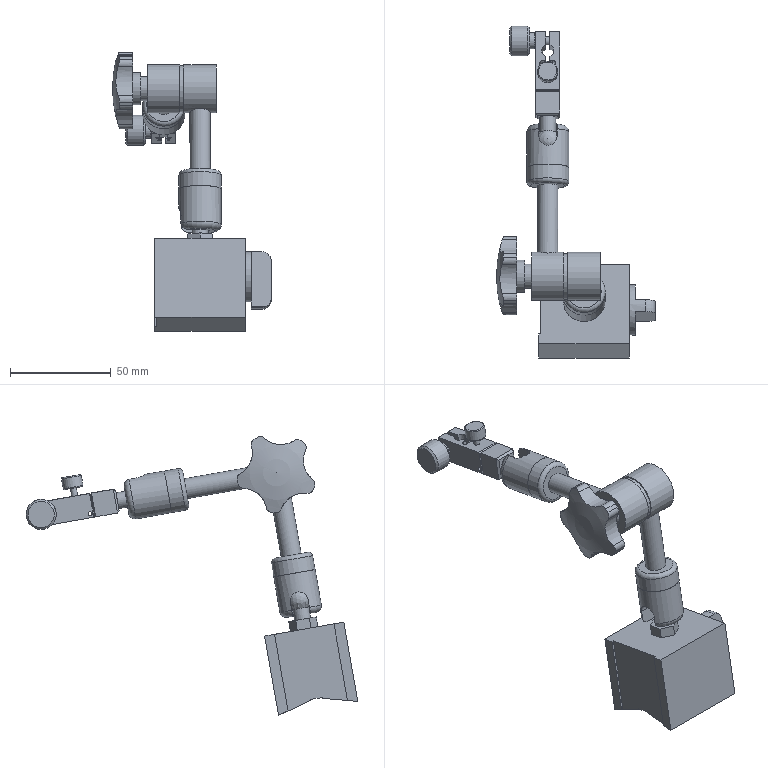Assembly | NX | mm | 16 component files | 16 solids | 236 faces | box 79 x 164.94 x 138.57 mm | volume 118951 mm3 | plane 127 | cylinder 82 | cone 17 | torus 7 | sphere 3 | commonest cylinder face diameters 6 x14 16 x11 24 x7 10 x6 40 x5 8 x5 3 x4 21 x4
Bill of materials:
unnamed part 1 | 1 |  | Rectangular block with chamfered edges, split by a narrow slot along its length; the slot runs through a large round hole and an obround pocket on the top face. There are cross-holes in the end faces and a notched channel on the underside.
unnamed part 2 | 1 |  | Pin made of a slender cylindrical shank and a larger cylindrical head. One side of the head has an angled flat cut, and both ends are chamfered.
unnamed part 3 | 2 |  | Thin-walled cylindrical sleeve/tube with a U-shaped notch cut into one end. The outer edge at the notched end is rounded.
unnamed part 4 | 1 |  | Ball stud: a sphere on a cylindrical neck, then a hexagonal collar, then a cylindrical shank with a chamfered end.
unnamed part 5 | 1 |  | Large short cylindrical disc head with rounded edges, and a smaller slender cylindrical pin sticking out from the centre of one face.
unnamed part 6 | 1 |  | Stepped cylindrical part with three diameters on one axis: a large cylinder with chamfered ends, a medium shoulder with a chamfer, and a long slender shaft.
unnamed part 7 | 1 |  | Roughly cubic block with a small hole on the top face and a stepped ledge along the bottom. A short boss on one face carries a flat tab with a rounded end.
unnamed part 8 | 2 |  | Stepped cylindrical bushing with a through bore: a larger-diameter flange section with a rounded edge, and a smaller-diameter section that has a small step/groove.
unnamed part 9 | 2 |  | Short cylindrical ring/eye with a through bore, with a slender cylindrical rod attached to its outer surface, perpendicular to the ring axis.
unnamed part 10 | 1 |  | Ball on a cylindrical neck, mounted on a rectangular block with a chamfered edge. A thin flat tab with a small round hole and a chamfered corner extends from the block.
unnamed part 11 | 1 |  | Thick cylindrical spacer/ring with a central through hole. One side has an angled planar cut near one end, which leaves an elliptical flat face.
unnamed part 12 | 1 |  | Five-lobed star-shaped knob with scalloped concave sides between rounded lobes. It has a two-step cylindrical hub on one side and a small central bore.
unnamed part 13 | 1 |  | Axisymmetric flanged disc/collar: a thin, large-diameter central flange with a smaller-diameter cylindrical hub on each face, both hubs with chamfered outer edges, and a central through bore along the axis.
Mates:
1. concentric | ball_joint_screw 1 edge | magnetic_base 1 edge
2. align lock | ball_joint_outer_sleeve 2 face | ball_joint_screw 1 face
3. align lock | swing_rod 2 face | ball_joint_outer_sleeve 2 face
4. concentric | swing_rod_ball_joint_base 2 edge | ball_joint_outer_sleeve 2 edge
5. touch align | ball_joint_screw 1 face | swing_rod 2 face
6. concentric | locking_shaft 1 edge | swing_rod 2 edge
7. align lock | middle_spacer 1 face | locking_shaft 1 face
8. touch align | middle_spacer 1 face | swing_rod 2 face
9. align lock | swing_rod 1 face | locking_shaft 1 face
10. touch align | swing_rod 1 face | middle_spacer 1 face
11. concentric | swing_rod_ball_joint_base 1 edge | ball_joint_outer_sleeve 1 edge
12. align lock | ball_joint_base 1 face | ball_joint_outer_sleeve 1 face
13. concentric | ball_joint_base 1 edge | ball_joint_outer_sleeve 1 edge
14. align lock | swing_rod_ball_joint_base 1 face | swing_rod 1 face
15. concentric | locking_sleeve 1 edge | middle_spacer 1 edge
16. concentric | handwheel 1 edge | locking_sleeve 1 edge
17. parallel | indicator_clamp_block 1 face | ball_joint_base 1 edge
18. parallel | indicator_clamp_block 1 face | ball_joint_base 1 face
19. concentric | indicator_clamp_block 1 edge | ball_joint_base 1 edge
20. concentric | 16 1 edge | indicator_clamp_block 1 edge
21. concentric | indicator_lock_handwheel 1 edge | indicator_clamp_block 1 edge